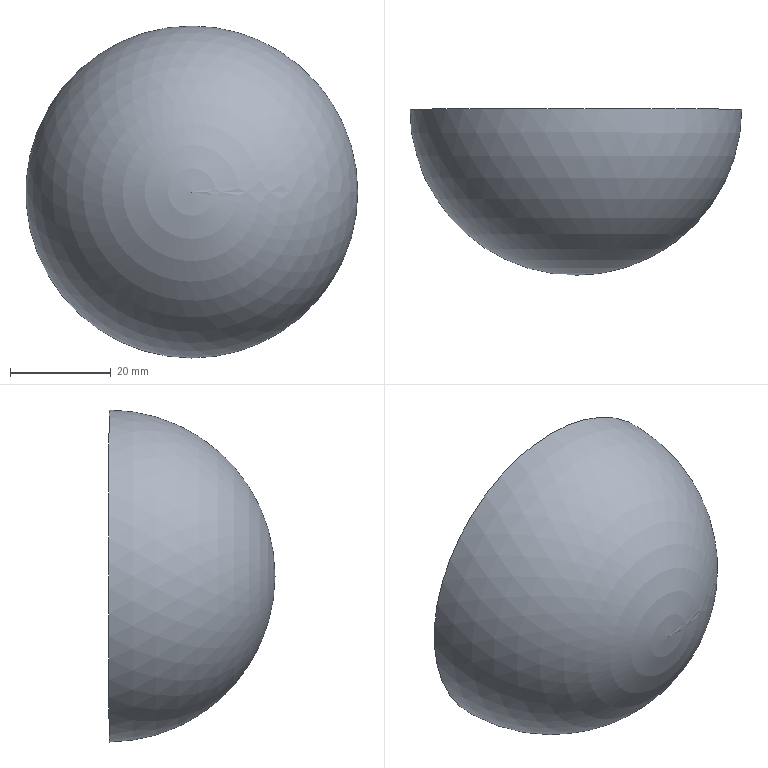Component | SolidWorks | RehabilitationChair-18-4-1 | 1 solid | 2 faces | box 65.75 x 32.87 x 65.75 mm | volume 74402 mm3 | plane 1 | sphere 1
STEP:
#1=COLOUR_RGB('',0.7922,0.8196,0.9333);
#2=FILL_AREA_STYLE_COLOUR('',#1);
#3=FILL_AREA_STYLE('',(#2));
#4=SURFACE_STYLE_FILL_AREA(#3);
#5=SURFACE_SIDE_STYLE('',(#4));
#6=SURFACE_STYLE_USAGE(.BOTH.,#5);
#7=PRESENTATION_STYLE_ASSIGNMENT((#6));
#8=CARTESIAN_POINT('',(-6.121,13.042,14.099));
#9=VERTEX_POINT('',#8);
#10=CARTESIAN_POINT('',(-6.121,13.042,16.687));
#11=VERTEX_POINT('',#10);
#12=CARTESIAN_POINT('',(-6.121,13.042,15.393));
#13=DIRECTION('',(0.00000124,1.,0.));
#14=DIRECTION('',(0.00000052,-0.,-1.));
#15=AXIS2_PLACEMENT_3D('',#12,#13,#14);
#16=CIRCLE('',#15,1.294);
#17=EDGE_CURVE('',#9,#11,#16,.T.);
#18=ORIENTED_EDGE('',*,*,#17,.T.);
#19=CARTESIAN_POINT('',(-6.121,13.042,15.393));
#20=DIRECTION('',(0.00000124,1.,0.));
#21=DIRECTION('',(0.00000052,-0.,-1.));
#22=AXIS2_PLACEMENT_3D('',#19,#20,#21);
#23=CIRCLE('',#22,1.294);
#24=EDGE_CURVE('',#11,#9,#23,.T.);
#25=ORIENTED_EDGE('',*,*,#24,.T.);
#26=EDGE_LOOP('',(#18,#25));
#27=FACE_OUTER_BOUND('',#26,.T.);
#28=CARTESIAN_POINT('',(-9.843,13.042,16.687));
#29=DIRECTION('',(-0.00000124,-1.,-0.));
#30=DIRECTION('',(0.00000052,-0.,-1.));
#31=AXIS2_PLACEMENT_3D('',#28,#29,#30);
#32=PLANE('',#31);
#33=ADVANCED_FACE('',(#27),#32,.F.);
#34=ORIENTED_EDGE('',*,*,#17,.F.);
#35=ORIENTED_EDGE('',*,*,#24,.F.);
#36=EDGE_LOOP('',(#34,#35));
#37=FACE_OUTER_BOUND('',#36,.T.);
#38=CARTESIAN_POINT('',(-6.121,13.042,15.393));
#39=DIRECTION('',(-0.00000124,-1.,-0.));
#40=DIRECTION('',(1.,-0.00000124,0.00000052));
#41=AXIS2_PLACEMENT_3D('',#38,#39,#40);
#42=SPHERICAL_SURFACE('',#41,1.294);
#43=ADVANCED_FACE('',(#37),#42,.T.);
#44=CLOSED_SHELL('',(#33,#43));
#45=MANIFOLD_SOLID_BREP('',#44);
#46=STYLED_ITEM('',(#7),#45);
#47=(LENGTH_UNIT()NAMED_UNIT(*)SI_UNIT($,.METRE.));
#48=LENGTH_MEASURE_WITH_UNIT(LENGTH_MEASURE(0.0254),#47);
#49=DIMENSIONAL_EXPONENTS(1.,0.,0.,0.,0.,0.,0.);
#50=(CONVERSION_BASED_UNIT('',#48)LENGTH_UNIT()NAMED_UNIT(#49));
#51=UNCERTAINTY_MEASURE_WITH_UNIT(LENGTH_MEASURE(0.00001),#50,'','');
#52=(NAMED_UNIT(*)PLANE_ANGLE_UNIT()SI_UNIT($,.RADIAN.));
#53=(NAMED_UNIT(*)SI_UNIT($,.STERADIAN.)SOLID_ANGLE_UNIT());
#54=(GEOMETRIC_REPRESENTATION_CONTEXT(3)GLOBAL_UNCERTAINTY_ASSIGNED_CONTEXT((#51))GLOBAL_UNIT_ASSIGNED_CONTEXT((#50,#52,#53))REPRESENTATION_CONTEXT('',''));
#55=MECHANICAL_DESIGN_GEOMETRIC_PRESENTATION_REPRESENTATION('',(#46),#54);
#56=CARTESIAN_POINT('',(0.,0.,0.));
#57=DIRECTION('',(0.,0.,1.));
#58=DIRECTION('',(1.,0.,0.));
#59=AXIS2_PLACEMENT_3D('',#56,#57,#58);
#60=(LENGTH_UNIT()NAMED_UNIT(*)SI_UNIT($,.METRE.));
#61=LENGTH_MEASURE_WITH_UNIT(LENGTH_MEASURE(0.0254),#60);
#62=DIMENSIONAL_EXPONENTS(1.,0.,0.,0.,0.,0.,0.);
#63=(CONVERSION_BASED_UNIT('',#61)LENGTH_UNIT()NAMED_UNIT(#62));
#64=UNCERTAINTY_MEASURE_WITH_UNIT(LENGTH_MEASURE(0.00001),#63,'','');
#65=(NAMED_UNIT(*)PLANE_ANGLE_UNIT()SI_UNIT($,.RADIAN.));
#66=(NAMED_UNIT(*)SI_UNIT($,.STERADIAN.)SOLID_ANGLE_UNIT());
#67=(GEOMETRIC_REPRESENTATION_CONTEXT(3)GLOBAL_UNCERTAINTY_ASSIGNED_CONTEXT((#64))GLOBAL_UNIT_ASSIGNED_CONTEXT((#63,#65,#66))REPRESENTATION_CONTEXT('',''));
#68=ADVANCED_BREP_SHAPE_REPRESENTATION('',(#45,#59),#67);
#69=PRESENTATION_LAYER_ASSIGNMENT('','',(#46));